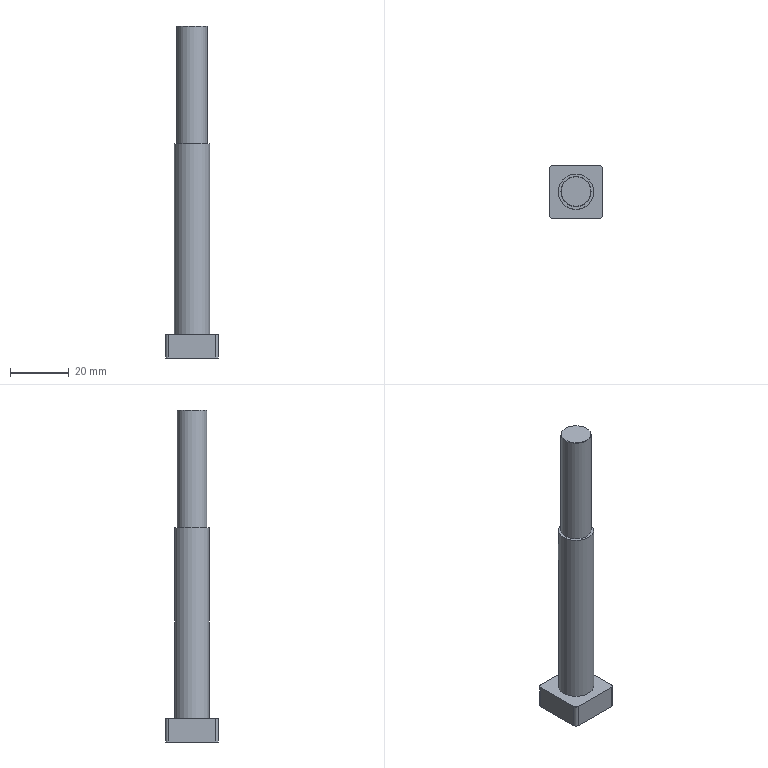Component | NX | 9_2 | 1 solid | 15 faces | box 18 x 18 x 113 mm | volume 13237 mm3 | plane 8 | cylinder 6 | cone 1 | commonest cylinder face diameters 2 x4 12 x1 10.25 x1
STEP:
#1=CARTESIAN_POINT('',(0.,0.,0.));
#2=DIRECTION('',(0.,0.,1.));
#3=DIRECTION('',(1.,0.,0.));
#4=AXIS2_PLACEMENT_3D('',#1,#2,#3);
#5=CARTESIAN_POINT('',(-38.,21.,-43.1));
#6=VERTEX_POINT('',#5);
#7=CARTESIAN_POINT('',(-22.,21.,-43.1));
#8=VERTEX_POINT('',#7);
#9=CARTESIAN_POINT('',(-38.,21.,-43.1));
#10=DIRECTION('',(1.,0.00000005,0.));
#11=VECTOR('',#10,1.);
#12=LINE('',#9,#11);
#13=CARTESIAN_POINT('',(-38.,21.,-51.1));
#14=DIRECTION('',(0.00000005,-1.,0.));
#15=DIRECTION('',(0.,0.,-1.));
#16=AXIS2_PLACEMENT_3D('',#13,#14,#15);
#17=PLANE('',#16);
#18=CARTESIAN_POINT('',(-8.,0.));
#19=DIRECTION('',(0.,1.));
#20=VECTOR('',#19,1.);
#21=LINE('',#18,#20);
#22=(GEOMETRIC_REPRESENTATION_CONTEXT(2)PARAMETRIC_REPRESENTATION_CONTEXT()REPRESENTATION_CONTEXT('',''));
#23=DEFINITIONAL_REPRESENTATION('',(#21),#22);
#24=PCURVE('',#17,#23);
#25=CARTESIAN_POINT('',(-22.,22.,-43.1));
#26=DIRECTION('',(0.,0.,1.));
#27=DIRECTION('',(-1.,-0.00000005,0.));
#28=AXIS2_PLACEMENT_3D('',#25,#26,#27);
#29=PLANE('',#28);
#30=CARTESIAN_POINT('',(16.,1.));
#31=DIRECTION('',(-1.,-0.));
#32=VECTOR('',#31,1.);
#33=LINE('',#30,#32);
#34=(GEOMETRIC_REPRESENTATION_CONTEXT(2)PARAMETRIC_REPRESENTATION_CONTEXT()REPRESENTATION_CONTEXT('',''));
#35=DEFINITIONAL_REPRESENTATION('',(#33),#34);
#36=PCURVE('',#29,#35);
#37=SURFACE_CURVE('',#12,(#24,#36),.PCURVE_S1.);
#38=EDGE_CURVE('',#6,#8,#37,.T.);
#39=ORIENTED_EDGE('',*,*,#38,.F.);
#40=CARTESIAN_POINT('',(-38.,21.,-51.1));
#41=VERTEX_POINT('',#40);
#42=CARTESIAN_POINT('',(-38.,21.,-51.1));
#43=DIRECTION('',(0.,0.,1.));
#44=VECTOR('',#43,1.);
#45=LINE('',#42,#44);
#46=CARTESIAN_POINT('',(0.,0.));
#47=DIRECTION('',(-1.,0.));
#48=VECTOR('',#47,1.);
#49=LINE('',#46,#48);
#50=(GEOMETRIC_REPRESENTATION_CONTEXT(2)PARAMETRIC_REPRESENTATION_CONTEXT()REPRESENTATION_CONTEXT('',''));
#51=DEFINITIONAL_REPRESENTATION('',(#49),#50);
#52=PCURVE('',#17,#51);
#53=CARTESIAN_POINT('',(-38.,22.,-51.1));
#54=DIRECTION('',(0.,0.,1.));
#55=DIRECTION('',(-1.,-0.00000005,0.));
#56=AXIS2_PLACEMENT_3D('',#53,#54,#55);
#57=CYLINDRICAL_SURFACE('',#56,1.);
#58=CARTESIAN_POINT('',(1.571,0.));
#59=DIRECTION('',(0.,1.));
#60=VECTOR('',#59,1.);
#61=LINE('',#58,#60);
#62=(GEOMETRIC_REPRESENTATION_CONTEXT(2)PARAMETRIC_REPRESENTATION_CONTEXT()REPRESENTATION_CONTEXT('',''));
#63=DEFINITIONAL_REPRESENTATION('',(#61),#62);
#64=PCURVE('',#57,#63);
#65=SURFACE_CURVE('',#45,(#52,#64),.PCURVE_S1.);
#66=EDGE_CURVE('',#41,#6,#65,.T.);
#67=ORIENTED_EDGE('',*,*,#66,.F.);
#68=CARTESIAN_POINT('',(-22.,21.,-51.1));
#69=VERTEX_POINT('',#68);
#70=CARTESIAN_POINT('',(-38.,21.,-51.1));
#71=DIRECTION('',(1.,0.00000005,0.));
#72=VECTOR('',#71,1.);
#73=LINE('',#70,#72);
#74=CARTESIAN_POINT('',(0.,0.));
#75=DIRECTION('',(0.,1.));
#76=VECTOR('',#75,1.);
#77=LINE('',#74,#76);
#78=(GEOMETRIC_REPRESENTATION_CONTEXT(2)PARAMETRIC_REPRESENTATION_CONTEXT()REPRESENTATION_CONTEXT('',''));
#79=DEFINITIONAL_REPRESENTATION('',(#77),#78);
#80=PCURVE('',#17,#79);
#81=CARTESIAN_POINT('',(-22.,22.,-51.1));
#82=DIRECTION('',(0.,0.,1.));
#83=DIRECTION('',(-1.,-0.00000005,0.));
#84=AXIS2_PLACEMENT_3D('',#81,#82,#83);
#85=PLANE('',#84);
#86=CARTESIAN_POINT('',(16.,1.));
#87=DIRECTION('',(-1.,-0.));
#88=VECTOR('',#87,1.);
#89=LINE('',#86,#88);
#90=(GEOMETRIC_REPRESENTATION_CONTEXT(2)PARAMETRIC_REPRESENTATION_CONTEXT()REPRESENTATION_CONTEXT('',''));
#91=DEFINITIONAL_REPRESENTATION('',(#89),#90);
#92=PCURVE('',#85,#91);
#93=SURFACE_CURVE('',#73,(#80,#92),.PCURVE_S1.);
#94=EDGE_CURVE('',#41,#69,#93,.T.);
#95=ORIENTED_EDGE('',*,*,#94,.T.);
#96=CARTESIAN_POINT('',(-22.,21.,-51.1));
#97=DIRECTION('',(0.,0.,1.));
#98=VECTOR('',#97,1.);
#99=LINE('',#96,#98);
#100=CARTESIAN_POINT('',(0.,16.));
#101=DIRECTION('',(-1.,0.));
#102=VECTOR('',#101,1.);
#103=LINE('',#100,#102);
#104=(GEOMETRIC_REPRESENTATION_CONTEXT(2)PARAMETRIC_REPRESENTATION_CONTEXT()REPRESENTATION_CONTEXT('',''));
#105=DEFINITIONAL_REPRESENTATION('',(#103),#104);
#106=PCURVE('',#17,#105);
#107=CARTESIAN_POINT('',(-22.,22.,-51.1));
#108=DIRECTION('',(0.,0.,1.));
#109=DIRECTION('',(-1.,-0.00000005,0.));
#110=AXIS2_PLACEMENT_3D('',#107,#108,#109);
#111=CYLINDRICAL_SURFACE('',#110,1.);
#112=CARTESIAN_POINT('',(1.571,0.));
#113=DIRECTION('',(0.,1.));
#114=VECTOR('',#113,1.);
#115=LINE('',#112,#114);
#116=(GEOMETRIC_REPRESENTATION_CONTEXT(2)PARAMETRIC_REPRESENTATION_CONTEXT()REPRESENTATION_CONTEXT('',''));
#117=DEFINITIONAL_REPRESENTATION('',(#115),#116);
#118=PCURVE('',#111,#117);
#119=SURFACE_CURVE('',#99,(#106,#118),.PCURVE_S1.);
#120=EDGE_CURVE('',#69,#8,#119,.T.);
#121=ORIENTED_EDGE('',*,*,#120,.T.);
#122=EDGE_LOOP('',(#39,#67,#95,#121));
#123=FACE_BOUND('',#122,.T.);
#124=ADVANCED_FACE('',(#123),#17,.T.);
#125=CARTESIAN_POINT('',(-21.,22.,-43.1));
#126=VERTEX_POINT('',#125);
#127=CARTESIAN_POINT('',(-22.,22.,-43.1));
#128=DIRECTION('',(0.,0.,1.));
#129=DIRECTION('',(1.,0.00000005,0.));
#130=AXIS2_PLACEMENT_3D('',#127,#128,#129);
#131=CIRCLE('',#130,1.);
#132=CARTESIAN_POINT('',(-3.142,8.));
#133=DIRECTION('',(1.,0.));
#134=VECTOR('',#133,1.);
#135=LINE('',#132,#134);
#136=(GEOMETRIC_REPRESENTATION_CONTEXT(2)PARAMETRIC_REPRESENTATION_CONTEXT()REPRESENTATION_CONTEXT('',''));
#137=DEFINITIONAL_REPRESENTATION('',(#135),#136);
#138=PCURVE('',#111,#137);
#139=CARTESIAN_POINT('',(0.,0.));
#140=DIRECTION('',(-1.,-0.));
#141=AXIS2_PLACEMENT_2D('',#139,#140);
#142=CIRCLE('',#141,1.);
#143=(GEOMETRIC_REPRESENTATION_CONTEXT(2)PARAMETRIC_REPRESENTATION_CONTEXT()REPRESENTATION_CONTEXT('',''));
#144=DEFINITIONAL_REPRESENTATION('',(#142),#143);
#145=PCURVE('',#29,#144);
#146=SURFACE_CURVE('',#131,(#138,#145),.PCURVE_S1.);
#147=EDGE_CURVE('',#8,#126,#146,.T.);
#148=ORIENTED_EDGE('',*,*,#147,.F.);
#149=ORIENTED_EDGE('',*,*,#120,.F.);
#150=CARTESIAN_POINT('',(-21.,22.,-51.1));
#151=VERTEX_POINT('',#150);
#152=CARTESIAN_POINT('',(-22.,22.,-51.1));
#153=DIRECTION('',(0.,0.,1.));
#154=DIRECTION('',(1.,0.00000005,0.));
#155=AXIS2_PLACEMENT_3D('',#152,#153,#154);
#156=CIRCLE('',#155,1.);
#157=CARTESIAN_POINT('',(-3.142,0.));
#158=DIRECTION('',(1.,0.));
#159=VECTOR('',#158,1.);
#160=LINE('',#157,#159);
#161=(GEOMETRIC_REPRESENTATION_CONTEXT(2)PARAMETRIC_REPRESENTATION_CONTEXT()REPRESENTATION_CONTEXT('',''));
#162=DEFINITIONAL_REPRESENTATION('',(#160),#161);
#163=PCURVE('',#111,#162);
#164=CARTESIAN_POINT('',(0.,0.));
#165=DIRECTION('',(-1.,-0.));
#166=AXIS2_PLACEMENT_2D('',#164,#165);
#167=CIRCLE('',#166,1.);
#168=(GEOMETRIC_REPRESENTATION_CONTEXT(2)PARAMETRIC_REPRESENTATION_CONTEXT()REPRESENTATION_CONTEXT('',''));
#169=DEFINITIONAL_REPRESENTATION('',(#167),#168);
#170=PCURVE('',#85,#169);
#171=SURFACE_CURVE('',#156,(#163,#170),.PCURVE_S1.);
#172=EDGE_CURVE('',#69,#151,#171,.T.);
#173=ORIENTED_EDGE('',*,*,#172,.T.);
#174=CARTESIAN_POINT('',(-21.,22.,-51.1));
#175=DIRECTION('',(0.,0.,1.));
#176=VECTOR('',#175,1.);
#177=LINE('',#174,#176);
#178=CARTESIAN_POINT('',(3.142,0.));
#179=DIRECTION('',(0.,1.));
#180=VECTOR('',#179,1.);
#181=LINE('',#178,#180);
#182=(GEOMETRIC_REPRESENTATION_CONTEXT(2)PARAMETRIC_REPRESENTATION_CONTEXT()REPRESENTATION_CONTEXT('',''));
#183=DEFINITIONAL_REPRESENTATION('',(#181),#182);
#184=PCURVE('',#111,#183);
#185=CARTESIAN_POINT('',(-21.,22.,-51.1));
#186=DIRECTION('',(1.,0.00000005,0.));
#187=DIRECTION('',(0.00000005,-1.,0.));
#188=AXIS2_PLACEMENT_3D('',#185,#186,#187);
#189=PLANE('',#188);
#190=CARTESIAN_POINT('',(0.,0.));
#191=DIRECTION('',(0.,-1.));
#192=VECTOR('',#191,1.);
#193=LINE('',#190,#192);
#194=(GEOMETRIC_REPRESENTATION_CONTEXT(2)PARAMETRIC_REPRESENTATION_CONTEXT()REPRESENTATION_CONTEXT('',''));
#195=DEFINITIONAL_REPRESENTATION('',(#193),#194);
#196=PCURVE('',#189,#195);
#197=SURFACE_CURVE('',#177,(#184,#196),.PCURVE_S1.);
#198=EDGE_CURVE('',#151,#126,#197,.T.);
#199=ORIENTED_EDGE('',*,*,#198,.T.);
#200=EDGE_LOOP('',(#148,#149,#173,#199));
#201=FACE_BOUND('',#200,.T.);
#202=ADVANCED_FACE('',(#201),#111,.T.);
#203=CARTESIAN_POINT('',(-21.,38.,-43.1));
#204=VERTEX_POINT('',#203);
#205=CARTESIAN_POINT('',(-21.,22.,-43.1));
#206=DIRECTION('',(-0.00000005,1.,0.));
#207=VECTOR('',#206,1.);
#208=LINE('',#205,#207);
#209=CARTESIAN_POINT('',(0.,-8.));
#210=DIRECTION('',(-1.,0.));
#211=VECTOR('',#210,1.);
#212=LINE('',#209,#211);
#213=(GEOMETRIC_REPRESENTATION_CONTEXT(2)PARAMETRIC_REPRESENTATION_CONTEXT()REPRESENTATION_CONTEXT('',''));
#214=DEFINITIONAL_REPRESENTATION('',(#212),#213);
#215=PCURVE('',#189,#214);
#216=CARTESIAN_POINT('',(-1.,0.));
#217=DIRECTION('',(-0.,-1.));
#218=VECTOR('',#217,1.);
#219=LINE('',#216,#218);
#220=(GEOMETRIC_REPRESENTATION_CONTEXT(2)PARAMETRIC_REPRESENTATION_CONTEXT()REPRESENTATION_CONTEXT('',''));
#221=DEFINITIONAL_REPRESENTATION('',(#219),#220);
#222=PCURVE('',#29,#221);
#223=SURFACE_CURVE('',#208,(#215,#222),.PCURVE_S1.);
#224=EDGE_CURVE('',#126,#204,#223,.T.);
#225=ORIENTED_EDGE('',*,*,#224,.F.);
#226=ORIENTED_EDGE('',*,*,#198,.F.);
#227=CARTESIAN_POINT('',(-21.,38.,-51.1));
#228=VERTEX_POINT('',#227);
#229=CARTESIAN_POINT('',(-21.,22.,-51.1));
#230=DIRECTION('',(-0.00000005,1.,0.));
#231=VECTOR('',#230,1.);
#232=LINE('',#229,#231);
#233=CARTESIAN_POINT('',(0.,0.));
#234=DIRECTION('',(-1.,0.));
#235=VECTOR('',#234,1.);
#236=LINE('',#233,#235);
#237=(GEOMETRIC_REPRESENTATION_CONTEXT(2)PARAMETRIC_REPRESENTATION_CONTEXT()REPRESENTATION_CONTEXT('',''));
#238=DEFINITIONAL_REPRESENTATION('',(#236),#237);
#239=PCURVE('',#189,#238);
#240=CARTESIAN_POINT('',(-1.,0.));
#241=DIRECTION('',(-0.,-1.));
#242=VECTOR('',#241,1.);
#243=LINE('',#240,#242);
#244=(GEOMETRIC_REPRESENTATION_CONTEXT(2)PARAMETRIC_REPRESENTATION_CONTEXT()REPRESENTATION_CONTEXT('',''));
#245=DEFINITIONAL_REPRESENTATION('',(#243),#244);
#246=PCURVE('',#85,#245);
#247=SURFACE_CURVE('',#232,(#239,#246),.PCURVE_S1.);
#248=EDGE_CURVE('',#151,#228,#247,.T.);
#249=ORIENTED_EDGE('',*,*,#248,.T.);
#250=CARTESIAN_POINT('',(-21.,38.,-51.1));
#251=DIRECTION('',(0.,0.,1.));
#252=VECTOR('',#251,1.);
#253=LINE('',#250,#252);
#254=CARTESIAN_POINT('',(-16.,0.));
#255=DIRECTION('',(0.,-1.));
#256=VECTOR('',#255,1.);
#257=LINE('',#254,#256);
#258=(GEOMETRIC_REPRESENTATION_CONTEXT(2)PARAMETRIC_REPRESENTATION_CONTEXT()REPRESENTATION_CONTEXT('',''));
#259=DEFINITIONAL_REPRESENTATION('',(#257),#258);
#260=PCURVE('',#189,#259);
#261=CARTESIAN_POINT('',(-22.,38.,-51.1));
#262=DIRECTION('',(0.,0.,1.));
#263=DIRECTION('',(-1.,-0.00000005,0.));
#264=AXIS2_PLACEMENT_3D('',#261,#262,#263);
#265=CYLINDRICAL_SURFACE('',#264,1.);
#266=CARTESIAN_POINT('',(3.142,0.));
#267=DIRECTION('',(0.,1.));
#268=VECTOR('',#267,1.);
#269=LINE('',#266,#268);
#270=(GEOMETRIC_REPRESENTATION_CONTEXT(2)PARAMETRIC_REPRESENTATION_CONTEXT()REPRESENTATION_CONTEXT('',''));
#271=DEFINITIONAL_REPRESENTATION('',(#269),#270);
#272=PCURVE('',#265,#271);
#273=SURFACE_CURVE('',#253,(#260,#272),.PCURVE_S1.);
#274=EDGE_CURVE('',#228,#204,#273,.T.);
#275=ORIENTED_EDGE('',*,*,#274,.T.);
#276=EDGE_LOOP('',(#225,#226,#249,#275));
#277=FACE_BOUND('',#276,.T.);
#278=ADVANCED_FACE('',(#277),#189,.T.);
#279=CARTESIAN_POINT('',(-22.,39.,-43.1));
#280=VERTEX_POINT('',#279);
#281=CARTESIAN_POINT('',(-22.,38.,-43.1));
#282=DIRECTION('',(0.,0.,1.));
#283=DIRECTION('',(1.,0.00000005,0.));
#284=AXIS2_PLACEMENT_3D('',#281,#282,#283);
#285=CIRCLE('',#284,1.);
#286=CARTESIAN_POINT('',(3.142,8.));
#287=DIRECTION('',(1.,0.));
#288=VECTOR('',#287,1.);
#289=LINE('',#286,#288);
#290=(GEOMETRIC_REPRESENTATION_CONTEXT(2)PARAMETRIC_REPRESENTATION_CONTEXT()REPRESENTATION_CONTEXT('',''));
#291=DEFINITIONAL_REPRESENTATION('',(#289),#290);
#292=PCURVE('',#265,#291);
#293=CARTESIAN_POINT('',(-0.,-16.));
#294=DIRECTION('',(-1.,0.));
#295=AXIS2_PLACEMENT_2D('',#293,#294);
#296=CIRCLE('',#295,1.);
#297=(GEOMETRIC_REPRESENTATION_CONTEXT(2)PARAMETRIC_REPRESENTATION_CONTEXT()REPRESENTATION_CONTEXT('',''));
#298=DEFINITIONAL_REPRESENTATION('',(#296),#297);
#299=PCURVE('',#29,#298);
#300=SURFACE_CURVE('',#285,(#292,#299),.PCURVE_S1.);
#301=EDGE_CURVE('',#204,#280,#300,.T.);
#302=ORIENTED_EDGE('',*,*,#301,.F.);
#303=ORIENTED_EDGE('',*,*,#274,.F.);
#304=CARTESIAN_POINT('',(-22.,39.,-51.1));
#305=VERTEX_POINT('',#304);
#306=CARTESIAN_POINT('',(-22.,38.,-51.1));
#307=DIRECTION('',(0.,0.,1.));
#308=DIRECTION('',(1.,0.00000005,0.));
#309=AXIS2_PLACEMENT_3D('',#306,#307,#308);
#310=CIRCLE('',#309,1.);
#311=CARTESIAN_POINT('',(3.142,0.));
#312=DIRECTION('',(1.,0.));
#313=VECTOR('',#312,1.);
#314=LINE('',#311,#313);
#315=(GEOMETRIC_REPRESENTATION_CONTEXT(2)PARAMETRIC_REPRESENTATION_CONTEXT()REPRESENTATION_CONTEXT('',''));
#316=DEFINITIONAL_REPRESENTATION('',(#314),#315);
#317=PCURVE('',#265,#316);
#318=CARTESIAN_POINT('',(-0.,-16.));
#319=DIRECTION('',(-1.,0.));
#320=AXIS2_PLACEMENT_2D('',#318,#319);
#321=CIRCLE('',#320,1.);
#322=(GEOMETRIC_REPRESENTATION_CONTEXT(2)PARAMETRIC_REPRESENTATION_CONTEXT()REPRESENTATION_CONTEXT('',''));
#323=DEFINITIONAL_REPRESENTATION('',(#321),#322);
#324=PCURVE('',#85,#323);
#325=SURFACE_CURVE('',#310,(#317,#324),.PCURVE_S1.);
#326=EDGE_CURVE('',#228,#305,#325,.T.);
#327=ORIENTED_EDGE('',*,*,#326,.T.);
#328=CARTESIAN_POINT('',(-22.,39.,-51.1));
#329=DIRECTION('',(0.,0.,1.));
#330=VECTOR('',#329,1.);
#331=LINE('',#328,#330);
#332=CARTESIAN_POINT('',(4.712,0.));
#333=DIRECTION('',(0.,1.));
#334=VECTOR('',#333,1.);
#335=LINE('',#332,#334);
#336=(GEOMETRIC_REPRESENTATION_CONTEXT(2)PARAMETRIC_REPRESENTATION_CONTEXT()REPRESENTATION_CONTEXT('',''));
#337=DEFINITIONAL_REPRESENTATION('',(#335),#336);
#338=PCURVE('',#265,#337);
#339=CARTESIAN_POINT('',(-22.,39.,-51.1));
#340=DIRECTION('',(-0.00000005,1.,0.));
#341=DIRECTION('',(1.,0.00000005,0.));
#342=AXIS2_PLACEMENT_3D('',#339,#340,#341);
#343=PLANE('',#342);
#344=CARTESIAN_POINT('',(0.,0.));
#345=DIRECTION('',(0.,-1.));
#346=VECTOR('',#345,1.);
#347=LINE('',#344,#346);
#348=(GEOMETRIC_REPRESENTATION_CONTEXT(2)PARAMETRIC_REPRESENTATION_CONTEXT()REPRESENTATION_CONTEXT('',''));
#349=DEFINITIONAL_REPRESENTATION('',(#347),#348);
#350=PCURVE('',#343,#349);
#351=SURFACE_CURVE('',#331,(#338,#350),.PCURVE_S1.);
#352=EDGE_CURVE('',#305,#280,#351,.T.);
#353=ORIENTED_EDGE('',*,*,#352,.T.);
#354=EDGE_LOOP('',(#302,#303,#327,#353));
#355=FACE_BOUND('',#354,.T.);
#356=ADVANCED_FACE('',(#355),#265,.T.);
#357=CARTESIAN_POINT('',(-38.,39.,-43.1));
#358=VERTEX_POINT('',#357);
#359=CARTESIAN_POINT('',(-22.,39.,-43.1));
#360=DIRECTION('',(-1.,-0.00000005,0.));
#361=VECTOR('',#360,1.);
#362=LINE('',#359,#361);
#363=CARTESIAN_POINT('',(0.,-8.));
#364=DIRECTION('',(-1.,0.));
#365=VECTOR('',#364,1.);
#366=LINE('',#363,#365);
#367=(GEOMETRIC_REPRESENTATION_CONTEXT(2)PARAMETRIC_REPRESENTATION_CONTEXT()REPRESENTATION_CONTEXT('',''));
#368=DEFINITIONAL_REPRESENTATION('',(#366),#367);
#369=PCURVE('',#343,#368);
#370=CARTESIAN_POINT('',(-0.,-17.));
#371=DIRECTION('',(1.,-0.));
#372=VECTOR('',#371,1.);
#373=LINE('',#370,#372);
#374=(GEOMETRIC_REPRESENTATION_CONTEXT(2)PARAMETRIC_REPRESENTATION_CONTEXT()REPRESENTATION_CONTEXT('',''));
#375=DEFINITIONAL_REPRESENTATION('',(#373),#374);
#376=PCURVE('',#29,#375);
#377=SURFACE_CURVE('',#362,(#369,#376),.PCURVE_S1.);
#378=EDGE_CURVE('',#280,#358,#377,.T.);
#379=ORIENTED_EDGE('',*,*,#378,.F.);
#380=ORIENTED_EDGE('',*,*,#352,.F.);
#381=CARTESIAN_POINT('',(-38.,39.,-51.1));
#382=VERTEX_POINT('',#381);
#383=CARTESIAN_POINT('',(-22.,39.,-51.1));
#384=DIRECTION('',(-1.,-0.00000005,0.));
#385=VECTOR('',#384,1.);
#386=LINE('',#383,#385);
#387=CARTESIAN_POINT('',(0.,0.));
#388=DIRECTION('',(-1.,0.));
#389=VECTOR('',#388,1.);
#390=LINE('',#387,#389);
#391=(GEOMETRIC_REPRESENTATION_CONTEXT(2)PARAMETRIC_REPRESENTATION_CONTEXT()REPRESENTATION_CONTEXT('',''));
#392=DEFINITIONAL_REPRESENTATION('',(#390),#391);
#393=PCURVE('',#343,#392);
#394=CARTESIAN_POINT('',(-0.,-17.));
#395=DIRECTION('',(1.,-0.));
#396=VECTOR('',#395,1.);
#397=LINE('',#394,#396);
#398=(GEOMETRIC_REPRESENTATION_CONTEXT(2)PARAMETRIC_REPRESENTATION_CONTEXT()REPRESENTATION_CONTEXT('',''));
#399=DEFINITIONAL_REPRESENTATION('',(#397),#398);
#400=PCURVE('',#85,#399);
#401=SURFACE_CURVE('',#386,(#393,#400),.PCURVE_S1.);
#402=EDGE_CURVE('',#305,#382,#401,.T.);
#403=ORIENTED_EDGE('',*,*,#402,.T.);
#404=CARTESIAN_POINT('',(-38.,39.,-51.1));
#405=DIRECTION('',(0.,0.,1.));
#406=VECTOR('',#405,1.);
#407=LINE('',#404,#406);
#408=CARTESIAN_POINT('',(-16.,0.));
#409=DIRECTION('',(0.,-1.));
#410=VECTOR('',#409,1.);
#411=LINE('',#408,#410);
#412=(GEOMETRIC_REPRESENTATION_CONTEXT(2)PARAMETRIC_REPRESENTATION_CONTEXT()REPRESENTATION_CONTEXT('',''));
#413=DEFINITIONAL_REPRESENTATION('',(#411),#412);
#414=PCURVE('',#343,#413);
#415=CARTESIAN_POINT('',(-38.,38.,-51.1));
#416=DIRECTION('',(0.,0.,1.));
#417=DIRECTION('',(-1.,-0.00000005,0.));
#418=AXIS2_PLACEMENT_3D('',#415,#416,#417);
#419=CYLINDRICAL_SURFACE('',#418,1.);
#420=CARTESIAN_POINT('',(4.712,0.));
#421=DIRECTION('',(0.,1.));
#422=VECTOR('',#421,1.);
#423=LINE('',#420,#422);
#424=(GEOMETRIC_REPRESENTATION_CONTEXT(2)PARAMETRIC_REPRESENTATION_CONTEXT()REPRESENTATION_CONTEXT('',''));
#425=DEFINITIONAL_REPRESENTATION('',(#423),#424);
#426=PCURVE('',#419,#425);
#427=SURFACE_CURVE('',#407,(#414,#426),.PCURVE_S1.);
#428=EDGE_CURVE('',#382,#358,#427,.T.);
#429=ORIENTED_EDGE('',*,*,#428,.T.);
#430=EDGE_LOOP('',(#379,#380,#403,#429));
#431=FACE_BOUND('',#430,.T.);
#432=ADVANCED_FACE('',(#431),#343,.T.);
#433=CARTESIAN_POINT('',(-39.,38.,-43.1));
#434=VERTEX_POINT('',#433);
#435=CARTESIAN_POINT('',(-38.,38.,-43.1));
#436=DIRECTION('',(0.,0.,1.));
#437=DIRECTION('',(1.,0.00000005,0.));
#438=AXIS2_PLACEMENT_3D('',#435,#436,#437);
#439=CIRCLE('',#438,1.);
#440=CARTESIAN_POINT('',(3.142,8.));
#441=DIRECTION('',(1.,0.));
#442=VECTOR('',#441,1.);
#443=LINE('',#440,#442);
#444=(GEOMETRIC_REPRESENTATION_CONTEXT(2)PARAMETRIC_REPRESENTATION_CONTEXT()REPRESENTATION_CONTEXT('',''));
#445=DEFINITIONAL_REPRESENTATION('',(#443),#444);
#446=PCURVE('',#419,#445);
#447=CARTESIAN_POINT('',(16.,-16.));
#448=DIRECTION('',(-1.,0.));
#449=AXIS2_PLACEMENT_2D('',#447,#448);
#450=CIRCLE('',#449,1.);
#451=(GEOMETRIC_REPRESENTATION_CONTEXT(2)PARAMETRIC_REPRESENTATION_CONTEXT()REPRESENTATION_CONTEXT('',''));
#452=DEFINITIONAL_REPRESENTATION('',(#450),#451);
#453=PCURVE('',#29,#452);
#454=SURFACE_CURVE('',#439,(#446,#453),.PCURVE_S1.);
#455=EDGE_CURVE('',#358,#434,#454,.T.);
#456=ORIENTED_EDGE('',*,*,#455,.F.);
#457=ORIENTED_EDGE('',*,*,#428,.F.);
#458=CARTESIAN_POINT('',(-39.,38.,-51.1));
#459=VERTEX_POINT('',#458);
#460=CARTESIAN_POINT('',(-38.,38.,-51.1));
#461=DIRECTION('',(0.,0.,1.));
#462=DIRECTION('',(1.,0.00000005,0.));
#463=AXIS2_PLACEMENT_3D('',#460,#461,#462);
#464=CIRCLE('',#463,1.);
#465=CARTESIAN_POINT('',(3.142,0.));
#466=DIRECTION('',(1.,0.));
#467=VECTOR('',#466,1.);
#468=LINE('',#465,#467);
#469=(GEOMETRIC_REPRESENTATION_CONTEXT(2)PARAMETRIC_REPRESENTATION_CONTEXT()REPRESENTATION_CONTEXT('',''));
#470=DEFINITIONAL_REPRESENTATION('',(#468),#469);
#471=PCURVE('',#419,#470);
#472=CARTESIAN_POINT('',(16.,-16.));
#473=DIRECTION('',(-1.,0.));
#474=AXIS2_PLACEMENT_2D('',#472,#473);
#475=CIRCLE('',#474,1.);
#476=(GEOMETRIC_REPRESENTATION_CONTEXT(2)PARAMETRIC_REPRESENTATION_CONTEXT()REPRESENTATION_CONTEXT('',''));
#477=DEFINITIONAL_REPRESENTATION('',(#475),#476);
#478=PCURVE('',#85,#477);
#479=SURFACE_CURVE('',#464,(#471,#478),.PCURVE_S1.);
#480=EDGE_CURVE('',#382,#459,#479,.T.);
#481=ORIENTED_EDGE('',*,*,#480,.T.);
#482=CARTESIAN_POINT('',(-39.,38.,-51.1));
#483=DIRECTION('',(0.,0.,1.));
#484=VECTOR('',#483,1.);
#485=LINE('',#482,#484);
#486=CARTESIAN_POINT('',(6.283,0.));
#487=DIRECTION('',(0.,1.));
#488=VECTOR('',#487,1.);
#489=LINE('',#486,#488);
#490=(GEOMETRIC_REPRESENTATION_CONTEXT(2)PARAMETRIC_REPRESENTATION_CONTEXT()REPRESENTATION_CONTEXT('',''));
#491=DEFINITIONAL_REPRESENTATION('',(#489),#490);
#492=PCURVE('',#419,#491);
#493=CARTESIAN_POINT('',(-39.,38.,-51.1));
#494=DIRECTION('',(-1.,-0.00000005,0.));
#495=DIRECTION('',(-0.00000005,1.,0.));
#496=AXIS2_PLACEMENT_3D('',#493,#494,#495);
#497=PLANE('',#496);
#498=CARTESIAN_POINT('',(0.,0.));
#499=DIRECTION('',(0.,-1.));
#500=VECTOR('',#499,1.);
#501=LINE('',#498,#500);
#502=(GEOMETRIC_REPRESENTATION_CONTEXT(2)PARAMETRIC_REPRESENTATION_CONTEXT()REPRESENTATION_CONTEXT('',''));
#503=DEFINITIONAL_REPRESENTATION('',(#501),#502);
#504=PCURVE('',#497,#503);
#505=SURFACE_CURVE('',#485,(#492,#504),.PCURVE_S1.);
#506=EDGE_CURVE('',#459,#434,#505,.T.);
#507=ORIENTED_EDGE('',*,*,#506,.T.);
#508=EDGE_LOOP('',(#456,#457,#481,#507));
#509=FACE_BOUND('',#508,.T.);
#510=ADVANCED_FACE('',(#509),#419,.T.);
#511=CARTESIAN_POINT('',(-39.,22.,-43.1));
#512=VERTEX_POINT('',#511);
#513=CARTESIAN_POINT('',(-39.,38.,-43.1));
#514=DIRECTION('',(0.00000005,-1.,0.));
#515=VECTOR('',#514,1.);
#516=LINE('',#513,#515);
#517=CARTESIAN_POINT('',(0.,-8.));
#518=DIRECTION('',(-1.,0.));
#519=VECTOR('',#518,1.);
#520=LINE('',#517,#519);
#521=(GEOMETRIC_REPRESENTATION_CONTEXT(2)PARAMETRIC_REPRESENTATION_CONTEXT()REPRESENTATION_CONTEXT('',''));
#522=DEFINITIONAL_REPRESENTATION('',(#520),#521);
#523=PCURVE('',#497,#522);
#524=CARTESIAN_POINT('',(17.,-16.));
#525=DIRECTION('',(0.,1.));
#526=VECTOR('',#525,1.);
#527=LINE('',#524,#526);
#528=(GEOMETRIC_REPRESENTATION_CONTEXT(2)PARAMETRIC_REPRESENTATION_CONTEXT()REPRESENTATION_CONTEXT('',''));
#529=DEFINITIONAL_REPRESENTATION('',(#527),#528);
#530=PCURVE('',#29,#529);
#531=SURFACE_CURVE('',#516,(#523,#530),.PCURVE_S1.);
#532=EDGE_CURVE('',#434,#512,#531,.T.);
#533=ORIENTED_EDGE('',*,*,#532,.F.);
#534=ORIENTED_EDGE('',*,*,#506,.F.);
#535=CARTESIAN_POINT('',(-39.,22.,-51.1));
#536=VERTEX_POINT('',#535);
#537=CARTESIAN_POINT('',(-39.,38.,-51.1));
#538=DIRECTION('',(0.00000005,-1.,0.));
#539=VECTOR('',#538,1.);
#540=LINE('',#537,#539);
#541=CARTESIAN_POINT('',(0.,0.));
#542=DIRECTION('',(-1.,0.));
#543=VECTOR('',#542,1.);
#544=LINE('',#541,#543);
#545=(GEOMETRIC_REPRESENTATION_CONTEXT(2)PARAMETRIC_REPRESENTATION_CONTEXT()REPRESENTATION_CONTEXT('',''));
#546=DEFINITIONAL_REPRESENTATION('',(#544),#545);
#547=PCURVE('',#497,#546);
#548=CARTESIAN_POINT('',(17.,-16.));
#549=DIRECTION('',(0.,1.));
#550=VECTOR('',#549,1.);
#551=LINE('',#548,#550);
#552=(GEOMETRIC_REPRESENTATION_CONTEXT(2)PARAMETRIC_REPRESENTATION_CONTEXT()REPRESENTATION_CONTEXT('',''));
#553=DEFINITIONAL_REPRESENTATION('',(#551),#552);
#554=PCURVE('',#85,#553);
#555=SURFACE_CURVE('',#540,(#547,#554),.PCURVE_S1.);
#556=EDGE_CURVE('',#459,#536,#555,.T.);
#557=ORIENTED_EDGE('',*,*,#556,.T.);
#558=CARTESIAN_POINT('',(-39.,22.,-51.1));
#559=DIRECTION('',(0.,0.,1.));
#560=VECTOR('',#559,1.);
#561=LINE('',#558,#560);
#562=CARTESIAN_POINT('',(-16.,0.));
#563=DIRECTION('',(0.,-1.));
#564=VECTOR('',#563,1.);
#565=LINE('',#562,#564);
#566=(GEOMETRIC_REPRESENTATION_CONTEXT(2)PARAMETRIC_REPRESENTATION_CONTEXT()REPRESENTATION_CONTEXT('',''));
#567=DEFINITIONAL_REPRESENTATION('',(#565),#566);
#568=PCURVE('',#497,#567);
#569=CARTESIAN_POINT('',(0.,0.));
#570=DIRECTION('',(0.,1.));
#571=VECTOR('',#570,1.);
#572=LINE('',#569,#571);
#573=(GEOMETRIC_REPRESENTATION_CONTEXT(2)PARAMETRIC_REPRESENTATION_CONTEXT()REPRESENTATION_CONTEXT('',''));
#574=DEFINITIONAL_REPRESENTATION('',(#572),#573);
#575=PCURVE('',#57,#574);
#576=SURFACE_CURVE('',#561,(#568,#575),.PCURVE_S1.);
#577=EDGE_CURVE('',#536,#512,#576,.T.);
#578=ORIENTED_EDGE('',*,*,#577,.T.);
#579=EDGE_LOOP('',(#533,#534,#557,#578));
#580=FACE_BOUND('',#579,.T.);
#581=ADVANCED_FACE('',(#580),#497,.T.);
#582=CARTESIAN_POINT('',(-38.,22.,-43.1));
#583=DIRECTION('',(0.,0.,1.));
#584=DIRECTION('',(1.,0.00000005,0.));
#585=AXIS2_PLACEMENT_3D('',#582,#583,#584);
#586=CIRCLE('',#585,1.);
#587=CARTESIAN_POINT('',(-3.142,8.));
#588=DIRECTION('',(1.,0.));
#589=VECTOR('',#588,1.);
#590=LINE('',#587,#589);
#591=(GEOMETRIC_REPRESENTATION_CONTEXT(2)PARAMETRIC_REPRESENTATION_CONTEXT()REPRESENTATION_CONTEXT('',''));
#592=DEFINITIONAL_REPRESENTATION('',(#590),#591);
#593=PCURVE('',#57,#592);
#594=CARTESIAN_POINT('',(16.,0.));
#595=DIRECTION('',(-1.,-0.));
#596=AXIS2_PLACEMENT_2D('',#594,#595);
#597=CIRCLE('',#596,1.);
#598=(GEOMETRIC_REPRESENTATION_CONTEXT(2)PARAMETRIC_REPRESENTATION_CONTEXT()REPRESENTATION_CONTEXT('',''));
#599=DEFINITIONAL_REPRESENTATION('',(#597),#598);
#600=PCURVE('',#29,#599);
#601=SURFACE_CURVE('',#586,(#593,#600),.PCURVE_S1.);
#602=EDGE_CURVE('',#512,#6,#601,.T.);
#603=ORIENTED_EDGE('',*,*,#602,.F.);
#604=ORIENTED_EDGE('',*,*,#577,.F.);
#605=CARTESIAN_POINT('',(-38.,22.,-51.1));
#606=DIRECTION('',(0.,0.,1.));
#607=DIRECTION('',(1.,0.00000005,0.));
#608=AXIS2_PLACEMENT_3D('',#605,#606,#607);
#609=CIRCLE('',#608,1.);
#610=CARTESIAN_POINT('',(-3.142,0.));
#611=DIRECTION('',(1.,0.));
#612=VECTOR('',#611,1.);
#613=LINE('',#610,#612);
#614=(GEOMETRIC_REPRESENTATION_CONTEXT(2)PARAMETRIC_REPRESENTATION_CONTEXT()REPRESENTATION_CONTEXT('',''));
#615=DEFINITIONAL_REPRESENTATION('',(#613),#614);
#616=PCURVE('',#57,#615);
#617=CARTESIAN_POINT('',(16.,0.));
#618=DIRECTION('',(-1.,-0.));
#619=AXIS2_PLACEMENT_2D('',#617,#618);
#620=CIRCLE('',#619,1.);
#621=(GEOMETRIC_REPRESENTATION_CONTEXT(2)PARAMETRIC_REPRESENTATION_CONTEXT()REPRESENTATION_CONTEXT('',''));
#622=DEFINITIONAL_REPRESENTATION('',(#620),#621);
#623=PCURVE('',#85,#622);
#624=SURFACE_CURVE('',#609,(#616,#623),.PCURVE_S1.);
#625=EDGE_CURVE('',#536,#41,#624,.T.);
#626=ORIENTED_EDGE('',*,*,#625,.T.);
#627=ORIENTED_EDGE('',*,*,#66,.T.);
#628=EDGE_LOOP('',(#603,#604,#626,#627));
#629=FACE_BOUND('',#628,.T.);
#630=ADVANCED_FACE('',(#629),#57,.T.);
#631=ORIENTED_EDGE('',*,*,#94,.F.);
#632=ORIENTED_EDGE('',*,*,#625,.F.);
#633=ORIENTED_EDGE('',*,*,#556,.F.);
#634=ORIENTED_EDGE('',*,*,#480,.F.);
#635=ORIENTED_EDGE('',*,*,#402,.F.);
#636=ORIENTED_EDGE('',*,*,#326,.F.);
#637=ORIENTED_EDGE('',*,*,#248,.F.);
#638=ORIENTED_EDGE('',*,*,#172,.F.);
#639=EDGE_LOOP('',(#631,#632,#633,#634,#635,#636,#637,#638));
#640=FACE_BOUND('',#639,.T.);
#641=ADVANCED_FACE('',(#640),#85,.F.);
#642=CARTESIAN_POINT('',(-24.,30.,-43.1));
#643=VERTEX_POINT('',#642);
#644=CARTESIAN_POINT('',(-30.,30.,-43.1));
#645=DIRECTION('',(0.,0.,1.));
#646=DIRECTION('',(1.,0.00000005,0.));
#647=AXIS2_PLACEMENT_3D('',#644,#645,#646);
#648=CIRCLE('',#647,6.);
#649=CARTESIAN_POINT('',(8.,-8.));
#650=DIRECTION('',(-1.,0.));
#651=AXIS2_PLACEMENT_2D('',#649,#650);
#652=CIRCLE('',#651,6.);
#653=(GEOMETRIC_REPRESENTATION_CONTEXT(2)PARAMETRIC_REPRESENTATION_CONTEXT()REPRESENTATION_CONTEXT('',''));
#654=DEFINITIONAL_REPRESENTATION('',(#652),#653);
#655=PCURVE('',#29,#654);
#656=CARTESIAN_POINT('',(-30.,30.,61.9));
#657=DIRECTION('',(0.,0.,-1.));
#658=DIRECTION('',(1.,0.00000005,0.));
#659=AXIS2_PLACEMENT_3D('',#656,#657,#658);
#660=CYLINDRICAL_SURFACE('',#659,6.);
#661=CARTESIAN_POINT('',(6.283,105.));
#662=DIRECTION('',(-1.,0.));
#663=VECTOR('',#662,1.);
#664=LINE('',#661,#663);
#665=(GEOMETRIC_REPRESENTATION_CONTEXT(2)PARAMETRIC_REPRESENTATION_CONTEXT()REPRESENTATION_CONTEXT('',''));
#666=DEFINITIONAL_REPRESENTATION('',(#664),#665);
#667=PCURVE('',#660,#666);
#668=SURFACE_CURVE('',#648,(#655,#667),.PCURVE_S1.);
#669=EDGE_CURVE('',#643,#643,#668,.T.);
#670=ORIENTED_EDGE('',*,*,#669,.F.);
#671=EDGE_LOOP('',(#670));
#672=FACE_BOUND('',#671,.T.);
#673=ORIENTED_EDGE('',*,*,#38,.T.);
#674=ORIENTED_EDGE('',*,*,#147,.T.);
#675=ORIENTED_EDGE('',*,*,#224,.T.);
#676=ORIENTED_EDGE('',*,*,#301,.T.);
#677=ORIENTED_EDGE('',*,*,#378,.T.);
#678=ORIENTED_EDGE('',*,*,#455,.T.);
#679=ORIENTED_EDGE('',*,*,#532,.T.);
#680=ORIENTED_EDGE('',*,*,#602,.T.);
#681=EDGE_LOOP('',(#673,#674,#675,#676,#677,#678,#679,#680));
#682=FACE_BOUND('',#681,.T.);
#683=ADVANCED_FACE('',(#672,#682),#29,.T.);
#684=CARTESIAN_POINT('',(-24.,30.,21.9));
#685=VERTEX_POINT('',#684);
#686=CARTESIAN_POINT('',(-30.,30.,21.9));
#687=DIRECTION('',(0.,0.,-1.));
#688=DIRECTION('',(1.,0.00000005,0.));
#689=AXIS2_PLACEMENT_3D('',#686,#687,#688);
#690=CIRCLE('',#689,6.);
#691=CARTESIAN_POINT('',(0.,40.));
#692=DIRECTION('',(1.,0.));
#693=VECTOR('',#692,1.);
#694=LINE('',#691,#693);
#695=(GEOMETRIC_REPRESENTATION_CONTEXT(2)PARAMETRIC_REPRESENTATION_CONTEXT()REPRESENTATION_CONTEXT('',''));
#696=DEFINITIONAL_REPRESENTATION('',(#694),#695);
#697=PCURVE('',#660,#696);
#698=CARTESIAN_POINT('',(-30.,30.,21.9));
#699=DIRECTION('',(0.,0.,-1.));
#700=DIRECTION('',(1.,0.00000005,0.));
#701=AXIS2_PLACEMENT_3D('',#698,#699,#700);
#702=PLANE('',#701);
#703=CARTESIAN_POINT('',(0.,0.));
#704=DIRECTION('',(1.,0.));
#705=AXIS2_PLACEMENT_2D('',#703,#704);
#706=CIRCLE('',#705,6.);
#707=(GEOMETRIC_REPRESENTATION_CONTEXT(2)PARAMETRIC_REPRESENTATION_CONTEXT()REPRESENTATION_CONTEXT('',''));
#708=DEFINITIONAL_REPRESENTATION('',(#706),#707);
#709=PCURVE('',#702,#708);
#710=SURFACE_CURVE('',#690,(#697,#709),.PCURVE_S1.);
#711=EDGE_CURVE('',#685,#685,#710,.T.);
#712=ORIENTED_EDGE('',*,*,#711,.T.);
#713=CARTESIAN_POINT('',(-24.,30.,21.9));
#714=CARTESIAN_POINT('',(-24.,30.,-43.1));
#715=B_SPLINE_CURVE_WITH_KNOTS('',1,(#713,#714),.UNSPECIFIED.,.F.,.F.,(2,2),(40.,105.),.PIECEWISE_BEZIER_KNOTS.);
#716=CARTESIAN_POINT('',(6.283,0.));
#717=DIRECTION('',(0.,1.));
#718=VECTOR('',#717,1.);
#719=LINE('',#716,#718);
#720=(GEOMETRIC_REPRESENTATION_CONTEXT(2)PARAMETRIC_REPRESENTATION_CONTEXT()REPRESENTATION_CONTEXT('',''));
#721=DEFINITIONAL_REPRESENTATION('',(#719),#720);
#722=PCURVE('',#660,#721);
#723=CARTESIAN_POINT('',(0.,0.));
#724=DIRECTION('',(0.,1.));
#725=VECTOR('',#724,1.);
#726=LINE('',#723,#725);
#727=(GEOMETRIC_REPRESENTATION_CONTEXT(2)PARAMETRIC_REPRESENTATION_CONTEXT()REPRESENTATION_CONTEXT('',''));
#728=DEFINITIONAL_REPRESENTATION('',(#726),#727);
#729=PCURVE('',#660,#728);
#730=SEAM_CURVE('',#715,(#722,#729),.PCURVE_S1.);
#731=EDGE_CURVE('',#685,#643,#730,.T.);
#732=ORIENTED_EDGE('',*,*,#731,.T.);
#733=ORIENTED_EDGE('',*,*,#669,.T.);
#734=ORIENTED_EDGE('',*,*,#731,.F.);
#735=EDGE_LOOP('',(#712,#732,#733,#734));
#736=FACE_BOUND('',#735,.T.);
#737=ADVANCED_FACE('',(#736),#660,.T.);
#738=CARTESIAN_POINT('',(-24.875,30.,21.9));
#739=VERTEX_POINT('',#738);
#740=CARTESIAN_POINT('',(-30.,30.,21.9));
#741=DIRECTION('',(0.,0.,1.));
#742=DIRECTION('',(1.,0.00000005,0.));
#743=AXIS2_PLACEMENT_3D('',#740,#741,#742);
#744=CIRCLE('',#743,5.125);
#745=CARTESIAN_POINT('',(5.125,-0.));
#746=CARTESIAN_POINT('',(5.125,-8.877));
#747=CARTESIAN_POINT('',(-2.562,-4.438));
#748=CARTESIAN_POINT('',(-10.25,0.));
#749=CARTESIAN_POINT('',(-2.562,4.438));
#750=CARTESIAN_POINT('',(5.125,8.877));
#751=CARTESIAN_POINT('',(5.125,-0.));
#752=(BOUNDED_CURVE()B_SPLINE_CURVE(2,(#745,#746,#747,#748,#749,#750,#751),.UNSPECIFIED.,.T.,.F.)B_SPLINE_CURVE_WITH_KNOTS((1,2,2,2,2,1),(-2.094,0.,2.094,4.189,6.283,8.378),.UNSPECIFIED.)CURVE()GEOMETRIC_REPRESENTATION_ITEM()RATIONAL_B_SPLINE_CURVE((1.,0.5,1.,0.5,1.,0.5,1.))REPRESENTATION_ITEM(''));
#753=(GEOMETRIC_REPRESENTATION_CONTEXT(2)PARAMETRIC_REPRESENTATION_CONTEXT()REPRESENTATION_CONTEXT('',''));
#754=DEFINITIONAL_REPRESENTATION('',(#752),#753);
#755=PCURVE('',#702,#754);
#756=CARTESIAN_POINT('',(-30.,30.,62.9));
#757=DIRECTION('',(0.,0.,-1.));
#758=DIRECTION('',(1.,0.00000005,0.));
#759=AXIS2_PLACEMENT_3D('',#756,#757,#758);
#760=CYLINDRICAL_SURFACE('',#759,5.125);
#761=CARTESIAN_POINT('',(6.283,41.));
#762=DIRECTION('',(-1.,0.));
#763=VECTOR('',#762,1.);
#764=LINE('',#761,#763);
#765=(GEOMETRIC_REPRESENTATION_CONTEXT(2)PARAMETRIC_REPRESENTATION_CONTEXT()REPRESENTATION_CONTEXT('',''));
#766=DEFINITIONAL_REPRESENTATION('',(#764),#765);
#767=PCURVE('',#760,#766);
#768=SURFACE_CURVE('',#744,(#755,#767),.PCURVE_S1.);
#769=EDGE_CURVE('',#739,#739,#768,.T.);
#770=ORIENTED_EDGE('',*,*,#769,.F.);
#771=EDGE_LOOP('',(#770));
#772=FACE_BOUND('',#771,.T.);
#773=ORIENTED_EDGE('',*,*,#711,.F.);
#774=EDGE_LOOP('',(#773));
#775=FACE_BOUND('',#774,.T.);
#776=ADVANCED_FACE('',(#772,#775),#702,.F.);
#777=CARTESIAN_POINT('',(-24.875,30.,61.775));
#778=VERTEX_POINT('',#777);
#779=CARTESIAN_POINT('',(-30.,30.,61.775));
#780=DIRECTION('',(0.,0.,1.));
#781=DIRECTION('',(1.,0.00000005,0.));
#782=AXIS2_PLACEMENT_3D('',#779,#780,#781);
#783=CIRCLE('',#782,5.125);
#784=CARTESIAN_POINT('',(6.283,1.125));
#785=DIRECTION('',(-1.,0.));
#786=VECTOR('',#785,1.);
#787=LINE('',#784,#786);
#788=(GEOMETRIC_REPRESENTATION_CONTEXT(2)PARAMETRIC_REPRESENTATION_CONTEXT()REPRESENTATION_CONTEXT('',''));
#789=DEFINITIONAL_REPRESENTATION('',(#787),#788);
#790=PCURVE('',#760,#789);
#791=CARTESIAN_POINT('',(-30.,30.,61.9));
#792=DIRECTION('',(0.,0.,-1.));
#793=DIRECTION('',(1.,0.00000005,0.));
#794=AXIS2_PLACEMENT_3D('',#791,#792,#793);
#795=CONICAL_SURFACE('',#794,5.,0.7854);
#796=CARTESIAN_POINT('',(6.283,0.125));
#797=DIRECTION('',(-1.,0.));
#798=VECTOR('',#797,1.);
#799=LINE('',#796,#798);
#800=(GEOMETRIC_REPRESENTATION_CONTEXT(2)PARAMETRIC_REPRESENTATION_CONTEXT()REPRESENTATION_CONTEXT('',''));
#801=DEFINITIONAL_REPRESENTATION('',(#799),#800);
#802=PCURVE('',#795,#801);
#803=SURFACE_CURVE('',#783,(#790,#802),.PCURVE_S1.);
#804=EDGE_CURVE('',#778,#778,#803,.T.);
#805=ORIENTED_EDGE('',*,*,#804,.F.);
#806=CARTESIAN_POINT('',(-24.875,30.,61.775));
#807=CARTESIAN_POINT('',(-24.875,30.,21.9));
#808=B_SPLINE_CURVE_WITH_KNOTS('',1,(#806,#807),.UNSPECIFIED.,.F.,.F.,(2,2),(1.125,41.),.PIECEWISE_BEZIER_KNOTS.);
#809=CARTESIAN_POINT('',(6.283,0.));
#810=DIRECTION('',(0.,1.));
#811=VECTOR('',#810,1.);
#812=LINE('',#809,#811);
#813=(GEOMETRIC_REPRESENTATION_CONTEXT(2)PARAMETRIC_REPRESENTATION_CONTEXT()REPRESENTATION_CONTEXT('',''));
#814=DEFINITIONAL_REPRESENTATION('',(#812),#813);
#815=PCURVE('',#760,#814);
#816=CARTESIAN_POINT('',(0.,0.));
#817=DIRECTION('',(0.,1.));
#818=VECTOR('',#817,1.);
#819=LINE('',#816,#818);
#820=(GEOMETRIC_REPRESENTATION_CONTEXT(2)PARAMETRIC_REPRESENTATION_CONTEXT()REPRESENTATION_CONTEXT('',''));
#821=DEFINITIONAL_REPRESENTATION('',(#819),#820);
#822=PCURVE('',#760,#821);
#823=SEAM_CURVE('',#808,(#815,#822),.PCURVE_S1.);
#824=EDGE_CURVE('',#778,#739,#823,.T.);
#825=ORIENTED_EDGE('',*,*,#824,.T.);
#826=ORIENTED_EDGE('',*,*,#769,.T.);
#827=ORIENTED_EDGE('',*,*,#824,.F.);
#828=EDGE_LOOP('',(#805,#825,#826,#827));
#829=FACE_BOUND('',#828,.T.);
#830=ADVANCED_FACE('',(#829),#760,.T.);
#831=CARTESIAN_POINT('',(-35.,30.,61.9));
#832=VERTEX_POINT('',#831);
#833=CARTESIAN_POINT('',(-25.,30.,61.9));
#834=VERTEX_POINT('',#833);
#835=CARTESIAN_POINT('',(-30.,30.,61.9));
#836=DIRECTION('',(0.,0.,1.));
#837=DIRECTION('',(-1.,-0.00000005,0.));
#838=AXIS2_PLACEMENT_3D('',#835,#836,#837);
#839=CIRCLE('',#838,5.);
#840=CARTESIAN_POINT('',(-30.,30.,61.9));
#841=DIRECTION('',(0.,0.,1.));
#842=DIRECTION('',(-1.,-0.00000005,0.));
#843=AXIS2_PLACEMENT_3D('',#840,#841,#842);
#844=PLANE('',#843);
#845=CARTESIAN_POINT('',(0.,0.));
#846=DIRECTION('',(1.,0.));
#847=AXIS2_PLACEMENT_2D('',#845,#846);
#848=CIRCLE('',#847,5.);
#849=(GEOMETRIC_REPRESENTATION_CONTEXT(2)PARAMETRIC_REPRESENTATION_CONTEXT()REPRESENTATION_CONTEXT('',''));
#850=DEFINITIONAL_REPRESENTATION('',(#848),#849);
#851=PCURVE('',#844,#850);
#852=CARTESIAN_POINT('',(3.142,0.));
#853=DIRECTION('',(-1.,0.));
#854=VECTOR('',#853,1.);
#855=LINE('',#852,#854);
#856=(GEOMETRIC_REPRESENTATION_CONTEXT(2)PARAMETRIC_REPRESENTATION_CONTEXT()REPRESENTATION_CONTEXT('',''));
#857=DEFINITIONAL_REPRESENTATION('',(#855),#856);
#858=PCURVE('',#795,#857);
#859=SURFACE_CURVE('',#839,(#851,#858),.PCURVE_S1.);
#860=EDGE_CURVE('',#832,#834,#859,.T.);
#861=ORIENTED_EDGE('',*,*,#860,.T.);
#862=CARTESIAN_POINT('',(-30.,30.,61.9));
#863=DIRECTION('',(0.,0.,1.));
#864=DIRECTION('',(-1.,-0.00000005,0.));
#865=AXIS2_PLACEMENT_3D('',#862,#863,#864);
#866=CIRCLE('',#865,5.);
#867=CARTESIAN_POINT('',(0.,0.));
#868=DIRECTION('',(1.,0.));
#869=AXIS2_PLACEMENT_2D('',#867,#868);
#870=CIRCLE('',#869,5.);
#871=(GEOMETRIC_REPRESENTATION_CONTEXT(2)PARAMETRIC_REPRESENTATION_CONTEXT()REPRESENTATION_CONTEXT('',''));
#872=DEFINITIONAL_REPRESENTATION('',(#870),#871);
#873=PCURVE('',#844,#872);
#874=CARTESIAN_POINT('',(9.425,0.));
#875=DIRECTION('',(-1.,0.));
#876=VECTOR('',#875,1.);
#877=LINE('',#874,#876);
#878=(GEOMETRIC_REPRESENTATION_CONTEXT(2)PARAMETRIC_REPRESENTATION_CONTEXT()REPRESENTATION_CONTEXT('',''));
#879=DEFINITIONAL_REPRESENTATION('',(#877),#878);
#880=PCURVE('',#795,#879);
#881=SURFACE_CURVE('',#866,(#873,#880),.PCURVE_S1.);
#882=EDGE_CURVE('',#834,#832,#881,.T.);
#883=ORIENTED_EDGE('',*,*,#882,.T.);
#884=EDGE_LOOP('',(#861,#883));
#885=FACE_BOUND('',#884,.T.);
#886=ADVANCED_FACE('',(#885),#844,.T.);
#887=ORIENTED_EDGE('',*,*,#882,.F.);
#888=CARTESIAN_POINT('',(-25.,30.,61.9));
#889=CARTESIAN_POINT('',(-24.875,30.,61.775));
#890=B_SPLINE_CURVE_WITH_KNOTS('',1,(#888,#889),.UNSPECIFIED.,.F.,.F.,(2,2),(0.,0.1768),.PIECEWISE_BEZIER_KNOTS.);
#891=CARTESIAN_POINT('',(6.283,0.));
#892=DIRECTION('',(0.,1.));
#893=VECTOR('',#892,1.);
#894=LINE('',#891,#893);
#895=(GEOMETRIC_REPRESENTATION_CONTEXT(2)PARAMETRIC_REPRESENTATION_CONTEXT()REPRESENTATION_CONTEXT('',''));
#896=DEFINITIONAL_REPRESENTATION('',(#894),#895);
#897=PCURVE('',#795,#896);
#898=CARTESIAN_POINT('',(0.,0.));
#899=DIRECTION('',(0.,1.));
#900=VECTOR('',#899,1.);
#901=LINE('',#898,#900);
#902=(GEOMETRIC_REPRESENTATION_CONTEXT(2)PARAMETRIC_REPRESENTATION_CONTEXT()REPRESENTATION_CONTEXT('',''));
#903=DEFINITIONAL_REPRESENTATION('',(#901),#902);
#904=PCURVE('',#795,#903);
#905=SEAM_CURVE('',#890,(#897,#904),.PCURVE_S1.);
#906=EDGE_CURVE('',#834,#778,#905,.T.);
#907=ORIENTED_EDGE('',*,*,#906,.T.);
#908=ORIENTED_EDGE('',*,*,#804,.T.);
#909=ORIENTED_EDGE('',*,*,#906,.F.);
#910=ORIENTED_EDGE('',*,*,#860,.F.);
#911=EDGE_LOOP('',(#887,#907,#908,#909,#910));
#912=FACE_BOUND('',#911,.T.);
#913=ADVANCED_FACE('',(#912),#795,.T.);
#914=CLOSED_SHELL('',(#124,#202,#278,#356,#432,#510,#581,#630,#641,#683,#737,#776,#830,#886,#913));
#915=MANIFOLD_SOLID_BREP('',#914);
#916=(LENGTH_UNIT()NAMED_UNIT(*)SI_UNIT(.MILLI.,.METRE.));
#917=UNCERTAINTY_MEASURE_WITH_UNIT(LENGTH_MEASURE(0.000002),#916,'','');
#918=(NAMED_UNIT(*)PLANE_ANGLE_UNIT()SI_UNIT($,.RADIAN.));
#919=(NAMED_UNIT(*)SI_UNIT($,.STERADIAN.)SOLID_ANGLE_UNIT());
#920=(GEOMETRIC_REPRESENTATION_CONTEXT(3)GLOBAL_UNCERTAINTY_ASSIGNED_CONTEXT((#917))GLOBAL_UNIT_ASSIGNED_CONTEXT((#916,#918,#919))REPRESENTATION_CONTEXT('',''));
#921=ADVANCED_BREP_SHAPE_REPRESENTATION('',(#4,#915),#920);